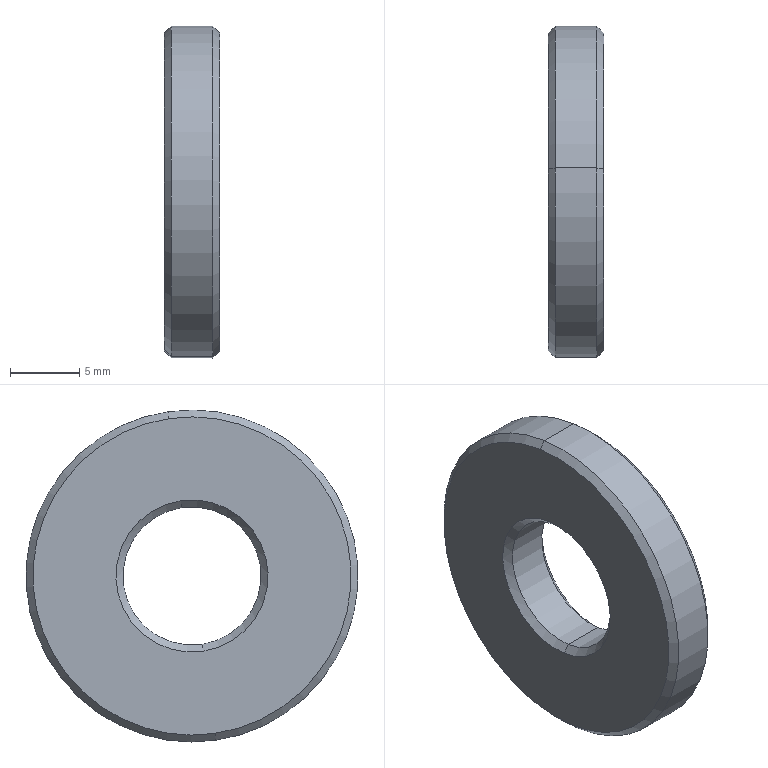Component | SolidWorks | Washer-4 | 1 solid | 14 faces | box 4 x 24 x 24 mm | volume 1469 mm3 | cone 8 | cylinder 4 | plane 2 | commonest cylinder face diameters 10 x2 24 x2
build123d program:
from build123d import *

# Parameters (mm, degrees)
SKETCH1_R           = 12
SKETCH1_R_2         = 5
BOSS_EXTRUDE1_DEPTH = 4
CHAMFER1_SIZE       = 0.5


with BuildPart() as part:
    # Sketch1 → Boss-Extrude1 (new body)
    with BuildSketch(Plane.XY):
        Circle(SKETCH1_R)
        Circle(SKETCH1_R_2, mode=Mode.SUBTRACT)
    extrude(amount=BOSS_EXTRUDE1_DEPTH)

    # Chamfer1
    chamfer1_edges = [part.edges().sort_by_distance(p)[0] for p in [
        (-12, 0, 0),
        (-12, 0, 4),
        (-5, 0, 0),
        (-5, 0, 4),
    ]]
    chamfer(chamfer1_edges, length=CHAMFER1_SIZE)


solid = part.part

# Placed as in the assembly
solid = solid.moved(Location((185.546, 77, 438.671), (0, 90, 0)))
STEP:
#1=COLOUR_RGB('',0.7922,0.8196,0.9333);
#2=FILL_AREA_STYLE_COLOUR('',#1);
#3=FILL_AREA_STYLE('',(#2));
#4=SURFACE_STYLE_FILL_AREA(#3);
#5=SURFACE_SIDE_STYLE('',(#4));
#6=SURFACE_STYLE_USAGE(.BOTH.,#5);
#7=PRESENTATION_STYLE_ASSIGNMENT((#6));
#8=CARTESIAN_POINT('',(7.462,2.966,16.822));
#9=VERTEX_POINT('',#8);
#10=CARTESIAN_POINT('',(7.462,3.097,17.719));
#11=VERTEX_POINT('',#10);
#12=CARTESIAN_POINT('',(7.462,3.031,17.271));
#13=DIRECTION('',(1.,0.,-0.));
#14=DIRECTION('',(-0.,-0.1438,-0.9896));
#15=AXIS2_PLACEMENT_3D('',#12,#13,#14);
#16=CIRCLE('',#15,0.4528);
#17=EDGE_CURVE('',#9,#11,#16,.T.);
#18=ORIENTED_EDGE('',*,*,#17,.F.);
#19=CARTESIAN_POINT('',(7.443,2.964,16.803));
#20=VERTEX_POINT('',#19);
#21=CARTESIAN_POINT('',(7.462,2.966,16.822));
#22=DIRECTION('',(-0.7071,-0.1017,-0.6998));
#23=VECTOR('',#22,39.37);
#24=LINE('',#21,#23);
#25=EDGE_CURVE('',#9,#20,#24,.T.);
#26=ORIENTED_EDGE('',*,*,#25,.T.);
#27=CARTESIAN_POINT('',(7.443,3.099,17.738));
#28=VERTEX_POINT('',#27);
#29=CARTESIAN_POINT('',(7.443,3.031,17.271));
#30=DIRECTION('',(-1.,-0.,0.));
#31=DIRECTION('',(-0.,-0.1438,-0.9896));
#32=AXIS2_PLACEMENT_3D('',#29,#30,#31);
#33=CIRCLE('',#32,0.4724);
#34=EDGE_CURVE('',#28,#20,#33,.T.);
#35=ORIENTED_EDGE('',*,*,#34,.F.);
#36=CARTESIAN_POINT('',(7.462,3.097,17.719));
#37=DIRECTION('',(-0.7071,0.1017,0.6998));
#38=VECTOR('',#37,39.37);
#39=LINE('',#36,#38);
#40=EDGE_CURVE('',#11,#28,#39,.T.);
#41=ORIENTED_EDGE('',*,*,#40,.F.);
#42=EDGE_LOOP('',(#18,#26,#35,#41));
#43=FACE_OUTER_BOUND('',#42,.T.);
#44=CARTESIAN_POINT('',(7.462,3.031,17.271));
#45=DIRECTION('',(-1.,-0.,0.));
#46=DIRECTION('',(0.,0.1438,0.9896));
#47=AXIS2_PLACEMENT_3D('',#44,#45,#46);
#48=CONICAL_SURFACE('',#47,0.4528,0.7854);
#49=ADVANCED_FACE('',(#43),#48,.T.);
#50=CARTESIAN_POINT('',(7.305,3.097,17.719));
#51=VERTEX_POINT('',#50);
#52=CARTESIAN_POINT('',(7.305,2.966,16.822));
#53=VERTEX_POINT('',#52);
#54=CARTESIAN_POINT('',(7.305,3.031,17.271));
#55=DIRECTION('',(-1.,-0.,0.));
#56=DIRECTION('',(-0.,-0.1438,-0.9896));
#57=AXIS2_PLACEMENT_3D('',#54,#55,#56);
#58=CIRCLE('',#57,0.4528);
#59=EDGE_CURVE('',#51,#53,#58,.T.);
#60=ORIENTED_EDGE('',*,*,#59,.F.);
#61=CARTESIAN_POINT('',(7.325,3.099,17.738));
#62=VERTEX_POINT('',#61);
#63=CARTESIAN_POINT('',(7.325,3.099,17.738));
#64=DIRECTION('',(0.7071,0.1017,0.6998));
#65=VECTOR('',#64,39.37);
#66=LINE('',#63,#65);
#67=EDGE_CURVE('',#51,#62,#66,.T.);
#68=ORIENTED_EDGE('',*,*,#67,.T.);
#69=CARTESIAN_POINT('',(7.325,2.964,16.803));
#70=VERTEX_POINT('',#69);
#71=CARTESIAN_POINT('',(7.325,3.031,17.271));
#72=DIRECTION('',(1.,0.,-0.));
#73=DIRECTION('',(-0.,-0.1438,-0.9896));
#74=AXIS2_PLACEMENT_3D('',#71,#72,#73);
#75=CIRCLE('',#74,0.4724);
#76=EDGE_CURVE('',#70,#62,#75,.T.);
#77=ORIENTED_EDGE('',*,*,#76,.F.);
#78=CARTESIAN_POINT('',(7.325,2.964,16.803));
#79=DIRECTION('',(0.7071,-0.1017,-0.6998));
#80=VECTOR('',#79,39.37);
#81=LINE('',#78,#80);
#82=EDGE_CURVE('',#53,#70,#81,.T.);
#83=ORIENTED_EDGE('',*,*,#82,.F.);
#84=EDGE_LOOP('',(#60,#68,#77,#83));
#85=FACE_OUTER_BOUND('',#84,.T.);
#86=CARTESIAN_POINT('',(7.325,3.031,17.271));
#87=DIRECTION('',(1.,0.,-0.));
#88=DIRECTION('',(-0.,-0.1438,-0.9896));
#89=AXIS2_PLACEMENT_3D('',#86,#87,#88);
#90=CONICAL_SURFACE('',#89,0.4724,0.7854);
#91=ADVANCED_FACE('',(#85),#90,.T.);
#92=CARTESIAN_POINT('',(7.443,3.06,17.465));
#93=VERTEX_POINT('',#92);
#94=CARTESIAN_POINT('',(7.443,3.003,17.076));
#95=VERTEX_POINT('',#94);
#96=CARTESIAN_POINT('',(7.443,3.031,17.271));
#97=DIRECTION('',(1.,0.,-0.));
#98=DIRECTION('',(-0.,-0.1438,-0.9896));
#99=AXIS2_PLACEMENT_3D('',#96,#97,#98);
#100=CIRCLE('',#99,0.1969);
#101=EDGE_CURVE('',#93,#95,#100,.T.);
#102=ORIENTED_EDGE('',*,*,#101,.F.);
#103=CARTESIAN_POINT('',(7.462,3.063,17.485));
#104=VERTEX_POINT('',#103);
#105=CARTESIAN_POINT('',(7.443,3.06,17.465));
#106=DIRECTION('',(0.7071,0.1017,0.6998));
#107=VECTOR('',#106,39.37);
#108=LINE('',#105,#107);
#109=EDGE_CURVE('',#93,#104,#108,.T.);
#110=ORIENTED_EDGE('',*,*,#109,.T.);
#111=CARTESIAN_POINT('',(7.462,3.,17.056));
#112=VERTEX_POINT('',#111);
#113=CARTESIAN_POINT('',(7.462,3.031,17.271));
#114=DIRECTION('',(-1.,-0.,0.));
#115=DIRECTION('',(-0.,-0.1438,-0.9896));
#116=AXIS2_PLACEMENT_3D('',#113,#114,#115);
#117=CIRCLE('',#116,0.2165);
#118=EDGE_CURVE('',#112,#104,#117,.T.);
#119=ORIENTED_EDGE('',*,*,#118,.F.);
#120=CARTESIAN_POINT('',(7.443,3.003,17.076));
#121=DIRECTION('',(0.7071,-0.1017,-0.6998));
#122=VECTOR('',#121,39.37);
#123=LINE('',#120,#122);
#124=EDGE_CURVE('',#95,#112,#123,.T.);
#125=ORIENTED_EDGE('',*,*,#124,.F.);
#126=EDGE_LOOP('',(#102,#110,#119,#125));
#127=FACE_OUTER_BOUND('',#126,.T.);
#128=CARTESIAN_POINT('',(7.443,3.031,17.271));
#129=DIRECTION('',(1.,0.,-0.));
#130=DIRECTION('',(-0.,-0.1438,-0.9896));
#131=AXIS2_PLACEMENT_3D('',#128,#129,#130);
#132=CONICAL_SURFACE('',#131,0.1969,0.7854);
#133=ADVANCED_FACE('',(#127),#132,.F.);
#134=CARTESIAN_POINT('',(7.325,3.003,17.076));
#135=VERTEX_POINT('',#134);
#136=CARTESIAN_POINT('',(7.325,3.06,17.465));
#137=VERTEX_POINT('',#136);
#138=CARTESIAN_POINT('',(7.325,3.031,17.271));
#139=DIRECTION('',(-1.,-0.,0.));
#140=DIRECTION('',(-0.,-0.1438,-0.9896));
#141=AXIS2_PLACEMENT_3D('',#138,#139,#140);
#142=CIRCLE('',#141,0.1969);
#143=EDGE_CURVE('',#135,#137,#142,.T.);
#144=ORIENTED_EDGE('',*,*,#143,.F.);
#145=CARTESIAN_POINT('',(7.305,3.,17.056));
#146=VERTEX_POINT('',#145);
#147=CARTESIAN_POINT('',(7.305,3.,17.056));
#148=DIRECTION('',(-0.7071,-0.1017,-0.6998));
#149=VECTOR('',#148,39.37);
#150=LINE('',#147,#149);
#151=EDGE_CURVE('',#135,#146,#150,.T.);
#152=ORIENTED_EDGE('',*,*,#151,.T.);
#153=CARTESIAN_POINT('',(7.305,3.063,17.485));
#154=VERTEX_POINT('',#153);
#155=CARTESIAN_POINT('',(7.305,3.031,17.271));
#156=DIRECTION('',(1.,0.,-0.));
#157=DIRECTION('',(-0.,-0.1438,-0.9896));
#158=AXIS2_PLACEMENT_3D('',#155,#156,#157);
#159=CIRCLE('',#158,0.2165);
#160=EDGE_CURVE('',#154,#146,#159,.T.);
#161=ORIENTED_EDGE('',*,*,#160,.F.);
#162=CARTESIAN_POINT('',(7.305,3.063,17.485));
#163=DIRECTION('',(-0.7071,0.1017,0.6998));
#164=VECTOR('',#163,39.37);
#165=LINE('',#162,#164);
#166=EDGE_CURVE('',#137,#154,#165,.T.);
#167=ORIENTED_EDGE('',*,*,#166,.F.);
#168=EDGE_LOOP('',(#144,#152,#161,#167));
#169=FACE_OUTER_BOUND('',#168,.T.);
#170=CARTESIAN_POINT('',(7.305,3.031,17.271));
#171=DIRECTION('',(-1.,-0.,0.));
#172=DIRECTION('',(0.,0.1438,0.9896));
#173=AXIS2_PLACEMENT_3D('',#170,#171,#172);
#174=CONICAL_SURFACE('',#173,0.2165,0.7854);
#175=ADVANCED_FACE('',(#169),#174,.F.);
#176=ORIENTED_EDGE('',*,*,#101,.T.);
#177=CARTESIAN_POINT('',(7.462,3.003,17.076));
#178=DIRECTION('',(-1.,-0.,0.));
#179=VECTOR('',#178,39.37);
#180=LINE('',#177,#179);
#181=EDGE_CURVE('',#95,#135,#180,.T.);
#182=ORIENTED_EDGE('',*,*,#181,.T.);
#183=ORIENTED_EDGE('',*,*,#143,.T.);
#184=CARTESIAN_POINT('',(7.462,3.06,17.465));
#185=DIRECTION('',(-1.,-0.,0.));
#186=VECTOR('',#185,39.37);
#187=LINE('',#184,#186);
#188=EDGE_CURVE('',#93,#137,#187,.T.);
#189=ORIENTED_EDGE('',*,*,#188,.F.);
#190=EDGE_LOOP('',(#176,#182,#183,#189));
#191=FACE_OUTER_BOUND('',#190,.T.);
#192=CARTESIAN_POINT('',(7.462,3.031,17.271));
#193=DIRECTION('',(-1.,-0.,0.));
#194=DIRECTION('',(0.,0.1438,0.9896));
#195=AXIS2_PLACEMENT_3D('',#192,#193,#194);
#196=CYLINDRICAL_SURFACE('',#195,0.1969);
#197=ADVANCED_FACE('',(#191),#196,.F.);
#198=ORIENTED_EDGE('',*,*,#34,.T.);
#199=CARTESIAN_POINT('',(7.462,2.964,16.803));
#200=DIRECTION('',(-1.,-0.,0.));
#201=VECTOR('',#200,39.37);
#202=LINE('',#199,#201);
#203=EDGE_CURVE('',#20,#70,#202,.T.);
#204=ORIENTED_EDGE('',*,*,#203,.T.);
#205=ORIENTED_EDGE('',*,*,#76,.T.);
#206=CARTESIAN_POINT('',(7.462,3.099,17.738));
#207=DIRECTION('',(-1.,-0.,0.));
#208=VECTOR('',#207,39.37);
#209=LINE('',#206,#208);
#210=EDGE_CURVE('',#28,#62,#209,.T.);
#211=ORIENTED_EDGE('',*,*,#210,.F.);
#212=EDGE_LOOP('',(#198,#204,#205,#211));
#213=FACE_OUTER_BOUND('',#212,.T.);
#214=CARTESIAN_POINT('',(7.462,3.031,17.271));
#215=DIRECTION('',(-1.,-0.,0.));
#216=DIRECTION('',(0.,0.1438,0.9896));
#217=AXIS2_PLACEMENT_3D('',#214,#215,#216);
#218=CYLINDRICAL_SURFACE('',#217,0.4724);
#219=ADVANCED_FACE('',(#213),#218,.T.);
#220=ORIENTED_EDGE('',*,*,#118,.T.);
#221=CARTESIAN_POINT('',(7.462,3.031,17.271));
#222=DIRECTION('',(-1.,-0.,0.));
#223=DIRECTION('',(-0.,-0.1438,-0.9896));
#224=AXIS2_PLACEMENT_3D('',#221,#222,#223);
#225=CIRCLE('',#224,0.2165);
#226=EDGE_CURVE('',#104,#112,#225,.T.);
#227=ORIENTED_EDGE('',*,*,#226,.T.);
#228=EDGE_LOOP('',(#220,#227));
#229=FACE_BOUND('',#228,.T.);
#230=CARTESIAN_POINT('',(7.462,3.031,17.271));
#231=DIRECTION('',(1.,0.,-0.));
#232=DIRECTION('',(-0.,-0.1438,-0.9896));
#233=AXIS2_PLACEMENT_3D('',#230,#231,#232);
#234=CIRCLE('',#233,0.4528);
#235=EDGE_CURVE('',#11,#9,#234,.T.);
#236=ORIENTED_EDGE('',*,*,#235,.T.);
#237=ORIENTED_EDGE('',*,*,#17,.T.);
#238=EDGE_LOOP('',(#236,#237));
#239=FACE_OUTER_BOUND('',#238,.T.);
#240=CARTESIAN_POINT('',(7.462,3.031,17.271));
#241=DIRECTION('',(1.,0.,-0.));
#242=DIRECTION('',(-0.,-0.1438,-0.9896));
#243=AXIS2_PLACEMENT_3D('',#240,#241,#242);
#244=PLANE('',#243);
#245=ADVANCED_FACE('',(#229,#239),#244,.T.);
#246=ORIENTED_EDGE('',*,*,#160,.T.);
#247=CARTESIAN_POINT('',(7.305,3.031,17.271));
#248=DIRECTION('',(1.,0.,-0.));
#249=DIRECTION('',(-0.,-0.1438,-0.9896));
#250=AXIS2_PLACEMENT_3D('',#247,#248,#249);
#251=CIRCLE('',#250,0.2165);
#252=EDGE_CURVE('',#146,#154,#251,.T.);
#253=ORIENTED_EDGE('',*,*,#252,.T.);
#254=EDGE_LOOP('',(#246,#253));
#255=FACE_BOUND('',#254,.T.);
#256=CARTESIAN_POINT('',(7.305,3.031,17.271));
#257=DIRECTION('',(-1.,-0.,0.));
#258=DIRECTION('',(-0.,-0.1438,-0.9896));
#259=AXIS2_PLACEMENT_3D('',#256,#257,#258);
#260=CIRCLE('',#259,0.4528);
#261=EDGE_CURVE('',#53,#51,#260,.T.);
#262=ORIENTED_EDGE('',*,*,#261,.T.);
#263=ORIENTED_EDGE('',*,*,#59,.T.);
#264=EDGE_LOOP('',(#262,#263));
#265=FACE_OUTER_BOUND('',#264,.T.);
#266=CARTESIAN_POINT('',(7.305,3.031,17.271));
#267=DIRECTION('',(1.,0.,-0.));
#268=DIRECTION('',(-0.,-0.1438,-0.9896));
#269=AXIS2_PLACEMENT_3D('',#266,#267,#268);
#270=PLANE('',#269);
#271=ADVANCED_FACE('',(#255,#265),#270,.F.);
#272=ORIENTED_EDGE('',*,*,#203,.F.);
#273=CARTESIAN_POINT('',(7.443,3.031,17.271));
#274=DIRECTION('',(-1.,-0.,0.));
#275=DIRECTION('',(-0.,-0.1438,-0.9896));
#276=AXIS2_PLACEMENT_3D('',#273,#274,#275);
#277=CIRCLE('',#276,0.4724);
#278=EDGE_CURVE('',#20,#28,#277,.T.);
#279=ORIENTED_EDGE('',*,*,#278,.T.);
#280=ORIENTED_EDGE('',*,*,#210,.T.);
#281=CARTESIAN_POINT('',(7.325,3.031,17.271));
#282=DIRECTION('',(1.,0.,-0.));
#283=DIRECTION('',(-0.,-0.1438,-0.9896));
#284=AXIS2_PLACEMENT_3D('',#281,#282,#283);
#285=CIRCLE('',#284,0.4724);
#286=EDGE_CURVE('',#62,#70,#285,.T.);
#287=ORIENTED_EDGE('',*,*,#286,.T.);
#288=EDGE_LOOP('',(#272,#279,#280,#287));
#289=FACE_OUTER_BOUND('',#288,.T.);
#290=CARTESIAN_POINT('',(7.462,3.031,17.271));
#291=DIRECTION('',(-1.,-0.,0.));
#292=DIRECTION('',(0.,0.1438,0.9896));
#293=AXIS2_PLACEMENT_3D('',#290,#291,#292);
#294=CYLINDRICAL_SURFACE('',#293,0.4724);
#295=ADVANCED_FACE('',(#289),#294,.T.);
#296=ORIENTED_EDGE('',*,*,#181,.F.);
#297=CARTESIAN_POINT('',(7.443,3.031,17.271));
#298=DIRECTION('',(1.,0.,-0.));
#299=DIRECTION('',(-0.,-0.1438,-0.9896));
#300=AXIS2_PLACEMENT_3D('',#297,#298,#299);
#301=CIRCLE('',#300,0.1969);
#302=EDGE_CURVE('',#95,#93,#301,.T.);
#303=ORIENTED_EDGE('',*,*,#302,.T.);
#304=ORIENTED_EDGE('',*,*,#188,.T.);
#305=CARTESIAN_POINT('',(7.325,3.031,17.271));
#306=DIRECTION('',(-1.,-0.,0.));
#307=DIRECTION('',(-0.,-0.1438,-0.9896));
#308=AXIS2_PLACEMENT_3D('',#305,#306,#307);
#309=CIRCLE('',#308,0.1969);
#310=EDGE_CURVE('',#137,#135,#309,.T.);
#311=ORIENTED_EDGE('',*,*,#310,.T.);
#312=EDGE_LOOP('',(#296,#303,#304,#311));
#313=FACE_OUTER_BOUND('',#312,.T.);
#314=CARTESIAN_POINT('',(7.462,3.031,17.271));
#315=DIRECTION('',(-1.,-0.,0.));
#316=DIRECTION('',(0.,0.1438,0.9896));
#317=AXIS2_PLACEMENT_3D('',#314,#315,#316);
#318=CYLINDRICAL_SURFACE('',#317,0.1969);
#319=ADVANCED_FACE('',(#313),#318,.F.);
#320=ORIENTED_EDGE('',*,*,#151,.F.);
#321=ORIENTED_EDGE('',*,*,#310,.F.);
#322=ORIENTED_EDGE('',*,*,#166,.T.);
#323=ORIENTED_EDGE('',*,*,#252,.F.);
#324=EDGE_LOOP('',(#320,#321,#322,#323));
#325=FACE_OUTER_BOUND('',#324,.T.);
#326=CARTESIAN_POINT('',(7.305,3.031,17.271));
#327=DIRECTION('',(-1.,-0.,0.));
#328=DIRECTION('',(0.,0.1438,0.9896));
#329=AXIS2_PLACEMENT_3D('',#326,#327,#328);
#330=CONICAL_SURFACE('',#329,0.2165,0.7854);
#331=ADVANCED_FACE('',(#325),#330,.F.);
#332=ORIENTED_EDGE('',*,*,#109,.F.);
#333=ORIENTED_EDGE('',*,*,#302,.F.);
#334=ORIENTED_EDGE('',*,*,#124,.T.);
#335=ORIENTED_EDGE('',*,*,#226,.F.);
#336=EDGE_LOOP('',(#332,#333,#334,#335));
#337=FACE_OUTER_BOUND('',#336,.T.);
#338=CARTESIAN_POINT('',(7.443,3.031,17.271));
#339=DIRECTION('',(1.,0.,-0.));
#340=DIRECTION('',(-0.,-0.1438,-0.9896));
#341=AXIS2_PLACEMENT_3D('',#338,#339,#340);
#342=CONICAL_SURFACE('',#341,0.1969,0.7854);
#343=ADVANCED_FACE('',(#337),#342,.F.);
#344=ORIENTED_EDGE('',*,*,#67,.F.);
#345=ORIENTED_EDGE('',*,*,#261,.F.);
#346=ORIENTED_EDGE('',*,*,#82,.T.);
#347=ORIENTED_EDGE('',*,*,#286,.F.);
#348=EDGE_LOOP('',(#344,#345,#346,#347));
#349=FACE_OUTER_BOUND('',#348,.T.);
#350=CARTESIAN_POINT('',(7.325,3.031,17.271));
#351=DIRECTION('',(1.,0.,-0.));
#352=DIRECTION('',(-0.,-0.1438,-0.9896));
#353=AXIS2_PLACEMENT_3D('',#350,#351,#352);
#354=CONICAL_SURFACE('',#353,0.4724,0.7854);
#355=ADVANCED_FACE('',(#349),#354,.T.);
#356=ORIENTED_EDGE('',*,*,#25,.F.);
#357=ORIENTED_EDGE('',*,*,#235,.F.);
#358=ORIENTED_EDGE('',*,*,#40,.T.);
#359=ORIENTED_EDGE('',*,*,#278,.F.);
#360=EDGE_LOOP('',(#356,#357,#358,#359));
#361=FACE_OUTER_BOUND('',#360,.T.);
#362=CARTESIAN_POINT('',(7.462,3.031,17.271));
#363=DIRECTION('',(-1.,-0.,0.));
#364=DIRECTION('',(0.,0.1438,0.9896));
#365=AXIS2_PLACEMENT_3D('',#362,#363,#364);
#366=CONICAL_SURFACE('',#365,0.4528,0.7854);
#367=ADVANCED_FACE('',(#361),#366,.T.);
#368=CLOSED_SHELL('',(#49,#91,#133,#175,#197,#219,#245,#271,#295,#319,#331,#343,#355,#367));
#369=MANIFOLD_SOLID_BREP('',#368);
#370=STYLED_ITEM('',(#7),#369);
#371=(LENGTH_UNIT()NAMED_UNIT(*)SI_UNIT($,.METRE.));
#372=LENGTH_MEASURE_WITH_UNIT(LENGTH_MEASURE(0.0254),#371);
#373=DIMENSIONAL_EXPONENTS(1.,0.,0.,0.,0.,0.,0.);
#374=(CONVERSION_BASED_UNIT('',#372)LENGTH_UNIT()NAMED_UNIT(#373));
#375=UNCERTAINTY_MEASURE_WITH_UNIT(LENGTH_MEASURE(0.00001),#374,'','');
#376=(NAMED_UNIT(*)PLANE_ANGLE_UNIT()SI_UNIT($,.RADIAN.));
#377=(NAMED_UNIT(*)SI_UNIT($,.STERADIAN.)SOLID_ANGLE_UNIT());
#378=(GEOMETRIC_REPRESENTATION_CONTEXT(3)GLOBAL_UNCERTAINTY_ASSIGNED_CONTEXT((#375))GLOBAL_UNIT_ASSIGNED_CONTEXT((#374,#376,#377))REPRESENTATION_CONTEXT('',''));
#379=MECHANICAL_DESIGN_GEOMETRIC_PRESENTATION_REPRESENTATION('',(#370),#378);
#380=CARTESIAN_POINT('',(0.,0.,0.));
#381=DIRECTION('',(0.,0.,1.));
#382=DIRECTION('',(1.,0.,0.));
#383=AXIS2_PLACEMENT_3D('',#380,#381,#382);
#384=(LENGTH_UNIT()NAMED_UNIT(*)SI_UNIT($,.METRE.));
#385=LENGTH_MEASURE_WITH_UNIT(LENGTH_MEASURE(0.0254),#384);
#386=DIMENSIONAL_EXPONENTS(1.,0.,0.,0.,0.,0.,0.);
#387=(CONVERSION_BASED_UNIT('',#385)LENGTH_UNIT()NAMED_UNIT(#386));
#388=UNCERTAINTY_MEASURE_WITH_UNIT(LENGTH_MEASURE(0.00001),#387,'','');
#389=(NAMED_UNIT(*)PLANE_ANGLE_UNIT()SI_UNIT($,.RADIAN.));
#390=(NAMED_UNIT(*)SI_UNIT($,.STERADIAN.)SOLID_ANGLE_UNIT());
#391=(GEOMETRIC_REPRESENTATION_CONTEXT(3)GLOBAL_UNCERTAINTY_ASSIGNED_CONTEXT((#388))GLOBAL_UNIT_ASSIGNED_CONTEXT((#387,#389,#390))REPRESENTATION_CONTEXT('',''));
#392=ADVANCED_BREP_SHAPE_REPRESENTATION('',(#369,#383),#391);
#393=PRESENTATION_LAYER_ASSIGNMENT('','',(#370));